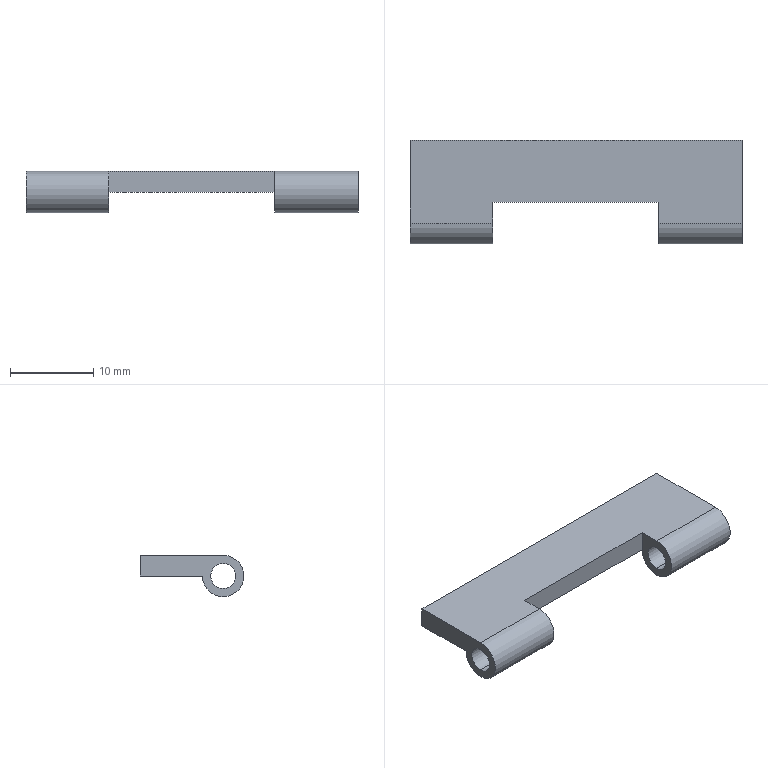Component | SolidWorks | ButtonStation-1_Hinge1-1 | 1 solid | 16 faces | box 40 x 12.5 x 5 mm | volume 1028 mm3 | cylinder 8 | plane 8 | commonest cylinder face diameters 5 x4 3 x4 | material Plain Carbon Steel
STEP:
#1=COLOUR_RGB('',0.7922,0.8196,0.9333);
#2=FILL_AREA_STYLE_COLOUR('',#1);
#3=FILL_AREA_STYLE('',(#2));
#4=SURFACE_STYLE_FILL_AREA(#3);
#5=SURFACE_SIDE_STYLE('',(#4));
#6=SURFACE_STYLE_USAGE(.BOTH.,#5);
#7=PRESENTATION_STYLE_ASSIGNMENT((#6));
#8=CARTESIAN_POINT('',(5.157,24.803,26.811));
#9=VERTEX_POINT('',#8);
#10=CARTESIAN_POINT('',(5.157,24.803,26.614));
#11=VERTEX_POINT('',#10);
#12=CARTESIAN_POINT('',(5.157,24.803,26.713));
#13=DIRECTION('',(1.,-0.,0.));
#14=DIRECTION('',(0.,0.,-1.));
#15=AXIS2_PLACEMENT_3D('',#12,#13,#14);
#16=CIRCLE('',#15,0.09843);
#17=EDGE_CURVE('',#9,#11,#16,.T.);
#18=ORIENTED_EDGE('',*,*,#17,.T.);
#19=CARTESIAN_POINT('',(5.551,24.803,26.614));
#20=VERTEX_POINT('',#19);
#21=CARTESIAN_POINT('',(5.157,24.803,26.614));
#22=DIRECTION('',(1.,-0.,0.));
#23=VECTOR('',#22,39.37);
#24=LINE('',#21,#23);
#25=EDGE_CURVE('',#11,#20,#24,.T.);
#26=ORIENTED_EDGE('',*,*,#25,.T.);
#27=CARTESIAN_POINT('',(5.551,24.803,26.811));
#28=VERTEX_POINT('',#27);
#29=CARTESIAN_POINT('',(5.551,24.803,26.713));
#30=DIRECTION('',(-1.,0.,-0.));
#31=DIRECTION('',(0.,0.,-1.));
#32=AXIS2_PLACEMENT_3D('',#29,#30,#31);
#33=CIRCLE('',#32,0.09843);
#34=EDGE_CURVE('',#20,#28,#33,.T.);
#35=ORIENTED_EDGE('',*,*,#34,.T.);
#36=CARTESIAN_POINT('',(5.157,24.803,26.811));
#37=DIRECTION('',(-1.,0.,-0.));
#38=VECTOR('',#37,39.37);
#39=LINE('',#36,#38);
#40=EDGE_CURVE('',#28,#9,#39,.T.);
#41=ORIENTED_EDGE('',*,*,#40,.T.);
#42=EDGE_LOOP('',(#18,#26,#35,#41));
#43=FACE_OUTER_BOUND('',#42,.T.);
#44=CARTESIAN_POINT('',(5.157,24.803,26.713));
#45=DIRECTION('',(1.,-0.,0.));
#46=DIRECTION('',(0.,0.,-1.));
#47=AXIS2_PLACEMENT_3D('',#44,#45,#46);
#48=CYLINDRICAL_SURFACE('',#47,0.09843);
#49=ADVANCED_FACE('',(#43),#48,.T.);
#50=CARTESIAN_POINT('',(6.339,24.803,26.811));
#51=VERTEX_POINT('',#50);
#52=CARTESIAN_POINT('',(6.339,24.803,26.614));
#53=VERTEX_POINT('',#52);
#54=CARTESIAN_POINT('',(6.339,24.803,26.713));
#55=DIRECTION('',(1.,-0.,0.));
#56=DIRECTION('',(0.,0.,-1.));
#57=AXIS2_PLACEMENT_3D('',#54,#55,#56);
#58=CIRCLE('',#57,0.09843);
#59=EDGE_CURVE('',#51,#53,#58,.T.);
#60=ORIENTED_EDGE('',*,*,#59,.T.);
#61=CARTESIAN_POINT('',(6.732,24.803,26.614));
#62=VERTEX_POINT('',#61);
#63=CARTESIAN_POINT('',(5.157,24.803,26.614));
#64=DIRECTION('',(1.,-0.,0.));
#65=VECTOR('',#64,39.37);
#66=LINE('',#63,#65);
#67=EDGE_CURVE('',#53,#62,#66,.T.);
#68=ORIENTED_EDGE('',*,*,#67,.T.);
#69=CARTESIAN_POINT('',(6.732,24.803,26.811));
#70=VERTEX_POINT('',#69);
#71=CARTESIAN_POINT('',(6.732,24.803,26.713));
#72=DIRECTION('',(-1.,0.,-0.));
#73=DIRECTION('',(0.,0.,-1.));
#74=AXIS2_PLACEMENT_3D('',#71,#72,#73);
#75=CIRCLE('',#74,0.09843);
#76=EDGE_CURVE('',#62,#70,#75,.T.);
#77=ORIENTED_EDGE('',*,*,#76,.T.);
#78=CARTESIAN_POINT('',(5.157,24.803,26.811));
#79=DIRECTION('',(-1.,0.,-0.));
#80=VECTOR('',#79,39.37);
#81=LINE('',#78,#80);
#82=EDGE_CURVE('',#70,#51,#81,.T.);
#83=ORIENTED_EDGE('',*,*,#82,.T.);
#84=EDGE_LOOP('',(#60,#68,#77,#83));
#85=FACE_OUTER_BOUND('',#84,.T.);
#86=CARTESIAN_POINT('',(5.157,24.803,26.713));
#87=DIRECTION('',(1.,-0.,0.));
#88=DIRECTION('',(0.,0.,-1.));
#89=AXIS2_PLACEMENT_3D('',#86,#87,#88);
#90=CYLINDRICAL_SURFACE('',#89,0.09843);
#91=ADVANCED_FACE('',(#85),#90,.T.);
#92=CARTESIAN_POINT('',(5.157,24.803,26.772));
#93=VERTEX_POINT('',#92);
#94=CARTESIAN_POINT('',(5.157,24.803,26.654));
#95=VERTEX_POINT('',#94);
#96=CARTESIAN_POINT('',(5.157,24.803,26.713));
#97=DIRECTION('',(1.,-0.,0.));
#98=DIRECTION('',(0.,0.,-1.));
#99=AXIS2_PLACEMENT_3D('',#96,#97,#98);
#100=CIRCLE('',#99,0.05906);
#101=EDGE_CURVE('',#93,#95,#100,.T.);
#102=ORIENTED_EDGE('',*,*,#101,.F.);
#103=CARTESIAN_POINT('',(5.551,24.803,26.772));
#104=VERTEX_POINT('',#103);
#105=CARTESIAN_POINT('',(5.157,24.803,26.772));
#106=DIRECTION('',(1.,-0.,0.));
#107=VECTOR('',#106,39.37);
#108=LINE('',#105,#107);
#109=EDGE_CURVE('',#93,#104,#108,.T.);
#110=ORIENTED_EDGE('',*,*,#109,.T.);
#111=CARTESIAN_POINT('',(5.551,24.803,26.654));
#112=VERTEX_POINT('',#111);
#113=CARTESIAN_POINT('',(5.551,24.803,26.713));
#114=DIRECTION('',(1.,-0.,0.));
#115=DIRECTION('',(0.,0.,-1.));
#116=AXIS2_PLACEMENT_3D('',#113,#114,#115);
#117=CIRCLE('',#116,0.05906);
#118=EDGE_CURVE('',#104,#112,#117,.T.);
#119=ORIENTED_EDGE('',*,*,#118,.T.);
#120=CARTESIAN_POINT('',(5.157,24.803,26.654));
#121=DIRECTION('',(1.,-0.,0.));
#122=VECTOR('',#121,39.37);
#123=LINE('',#120,#122);
#124=EDGE_CURVE('',#95,#112,#123,.T.);
#125=ORIENTED_EDGE('',*,*,#124,.F.);
#126=EDGE_LOOP('',(#102,#110,#119,#125));
#127=FACE_OUTER_BOUND('',#126,.T.);
#128=CARTESIAN_POINT('',(5.157,24.803,26.713));
#129=DIRECTION('',(1.,-0.,0.));
#130=DIRECTION('',(0.,0.,-1.));
#131=AXIS2_PLACEMENT_3D('',#128,#129,#130);
#132=CYLINDRICAL_SURFACE('',#131,0.05906);
#133=ADVANCED_FACE('',(#127),#132,.F.);
#134=CARTESIAN_POINT('',(6.339,24.803,26.654));
#135=VERTEX_POINT('',#134);
#136=CARTESIAN_POINT('',(6.339,24.803,26.772));
#137=VERTEX_POINT('',#136);
#138=CARTESIAN_POINT('',(6.339,24.803,26.713));
#139=DIRECTION('',(-1.,0.,-0.));
#140=DIRECTION('',(0.,0.,-1.));
#141=AXIS2_PLACEMENT_3D('',#138,#139,#140);
#142=CIRCLE('',#141,0.05906);
#143=EDGE_CURVE('',#135,#137,#142,.T.);
#144=ORIENTED_EDGE('',*,*,#143,.T.);
#145=CARTESIAN_POINT('',(6.732,24.803,26.772));
#146=VERTEX_POINT('',#145);
#147=CARTESIAN_POINT('',(5.157,24.803,26.772));
#148=DIRECTION('',(1.,-0.,0.));
#149=VECTOR('',#148,39.37);
#150=LINE('',#147,#149);
#151=EDGE_CURVE('',#137,#146,#150,.T.);
#152=ORIENTED_EDGE('',*,*,#151,.T.);
#153=CARTESIAN_POINT('',(6.732,24.803,26.654));
#154=VERTEX_POINT('',#153);
#155=CARTESIAN_POINT('',(6.732,24.803,26.713));
#156=DIRECTION('',(1.,-0.,0.));
#157=DIRECTION('',(0.,0.,-1.));
#158=AXIS2_PLACEMENT_3D('',#155,#156,#157);
#159=CIRCLE('',#158,0.05906);
#160=EDGE_CURVE('',#146,#154,#159,.T.);
#161=ORIENTED_EDGE('',*,*,#160,.T.);
#162=CARTESIAN_POINT('',(5.157,24.803,26.654));
#163=DIRECTION('',(1.,-0.,0.));
#164=VECTOR('',#163,39.37);
#165=LINE('',#162,#164);
#166=EDGE_CURVE('',#135,#154,#165,.T.);
#167=ORIENTED_EDGE('',*,*,#166,.F.);
#168=EDGE_LOOP('',(#144,#152,#161,#167));
#169=FACE_OUTER_BOUND('',#168,.T.);
#170=CARTESIAN_POINT('',(5.157,24.803,26.713));
#171=DIRECTION('',(1.,-0.,0.));
#172=DIRECTION('',(0.,0.,-1.));
#173=AXIS2_PLACEMENT_3D('',#170,#171,#172);
#174=CYLINDRICAL_SURFACE('',#173,0.05906);
#175=ADVANCED_FACE('',(#169),#174,.F.);
#176=CARTESIAN_POINT('',(5.551,24.902,26.811));
#177=VERTEX_POINT('',#176);
#178=CARTESIAN_POINT('',(5.551,24.932,26.811));
#179=DIRECTION('',(-0.,-1.,0.));
#180=VECTOR('',#179,39.37);
#181=LINE('',#178,#180);
#182=EDGE_CURVE('',#177,#28,#181,.T.);
#183=ORIENTED_EDGE('',*,*,#182,.F.);
#184=CARTESIAN_POINT('',(6.339,24.902,26.811));
#185=VERTEX_POINT('',#184);
#186=CARTESIAN_POINT('',(5.157,24.902,26.811));
#187=DIRECTION('',(-1.,0.,-0.));
#188=VECTOR('',#187,39.37);
#189=LINE('',#186,#188);
#190=EDGE_CURVE('',#185,#177,#189,.T.);
#191=ORIENTED_EDGE('',*,*,#190,.F.);
#192=CARTESIAN_POINT('',(6.339,24.932,26.811));
#193=DIRECTION('',(0.,1.,-0.));
#194=VECTOR('',#193,39.37);
#195=LINE('',#192,#194);
#196=EDGE_CURVE('',#51,#185,#195,.T.);
#197=ORIENTED_EDGE('',*,*,#196,.F.);
#198=ORIENTED_EDGE('',*,*,#82,.F.);
#199=CARTESIAN_POINT('',(6.732,25.197,26.811));
#200=VERTEX_POINT('',#199);
#201=CARTESIAN_POINT('',(6.732,24.932,26.811));
#202=DIRECTION('',(-0.,-1.,0.));
#203=VECTOR('',#202,39.37);
#204=LINE('',#201,#203);
#205=EDGE_CURVE('',#200,#70,#204,.T.);
#206=ORIENTED_EDGE('',*,*,#205,.F.);
#207=CARTESIAN_POINT('',(5.157,25.197,26.811));
#208=VERTEX_POINT('',#207);
#209=CARTESIAN_POINT('',(5.157,25.197,26.811));
#210=DIRECTION('',(1.,-0.,0.));
#211=VECTOR('',#210,39.37);
#212=LINE('',#209,#211);
#213=EDGE_CURVE('',#208,#200,#212,.T.);
#214=ORIENTED_EDGE('',*,*,#213,.F.);
#215=CARTESIAN_POINT('',(5.157,24.932,26.811));
#216=DIRECTION('',(0.,1.,-0.));
#217=VECTOR('',#216,39.37);
#218=LINE('',#215,#217);
#219=EDGE_CURVE('',#9,#208,#218,.T.);
#220=ORIENTED_EDGE('',*,*,#219,.F.);
#221=ORIENTED_EDGE('',*,*,#40,.F.);
#222=EDGE_LOOP('',(#183,#191,#197,#198,#206,#214,#220,#221));
#223=FACE_OUTER_BOUND('',#222,.T.);
#224=CARTESIAN_POINT('',(5.157,24.932,26.811));
#225=DIRECTION('',(0.,-0.,-1.));
#226=DIRECTION('',(-1.,0.,-0.));
#227=AXIS2_PLACEMENT_3D('',#224,#225,#226);
#228=PLANE('',#227);
#229=ADVANCED_FACE('',(#223),#228,.F.);
#230=ORIENTED_EDGE('',*,*,#25,.F.);
#231=CARTESIAN_POINT('',(5.157,24.902,26.713));
#232=VERTEX_POINT('',#231);
#233=CARTESIAN_POINT('',(5.157,24.803,26.713));
#234=DIRECTION('',(1.,-0.,0.));
#235=DIRECTION('',(0.,0.,-1.));
#236=AXIS2_PLACEMENT_3D('',#233,#234,#235);
#237=CIRCLE('',#236,0.09843);
#238=EDGE_CURVE('',#11,#232,#237,.T.);
#239=ORIENTED_EDGE('',*,*,#238,.T.);
#240=CARTESIAN_POINT('',(5.551,24.902,26.713));
#241=VERTEX_POINT('',#240);
#242=CARTESIAN_POINT('',(5.157,24.902,26.713));
#243=DIRECTION('',(1.,-0.,0.));
#244=VECTOR('',#243,39.37);
#245=LINE('',#242,#244);
#246=EDGE_CURVE('',#232,#241,#245,.T.);
#247=ORIENTED_EDGE('',*,*,#246,.T.);
#248=CARTESIAN_POINT('',(5.551,24.803,26.713));
#249=DIRECTION('',(-1.,0.,-0.));
#250=DIRECTION('',(0.,0.,-1.));
#251=AXIS2_PLACEMENT_3D('',#248,#249,#250);
#252=CIRCLE('',#251,0.09843);
#253=EDGE_CURVE('',#241,#20,#252,.T.);
#254=ORIENTED_EDGE('',*,*,#253,.T.);
#255=EDGE_LOOP('',(#230,#239,#247,#254));
#256=FACE_OUTER_BOUND('',#255,.T.);
#257=CARTESIAN_POINT('',(5.157,24.803,26.713));
#258=DIRECTION('',(1.,-0.,0.));
#259=DIRECTION('',(0.,0.,-1.));
#260=AXIS2_PLACEMENT_3D('',#257,#258,#259);
#261=CYLINDRICAL_SURFACE('',#260,0.09843);
#262=ADVANCED_FACE('',(#256),#261,.T.);
#263=CARTESIAN_POINT('',(5.551,24.803,26.713));
#264=DIRECTION('',(1.,-0.,0.));
#265=DIRECTION('',(0.,0.,-1.));
#266=AXIS2_PLACEMENT_3D('',#263,#264,#265);
#267=CIRCLE('',#266,0.05906);
#268=EDGE_CURVE('',#112,#104,#267,.T.);
#269=ORIENTED_EDGE('',*,*,#268,.F.);
#270=ORIENTED_EDGE('',*,*,#118,.F.);
#271=EDGE_LOOP('',(#269,#270));
#272=FACE_BOUND('',#271,.T.);
#273=ORIENTED_EDGE('',*,*,#253,.F.);
#274=CARTESIAN_POINT('',(5.551,24.902,26.614));
#275=DIRECTION('',(0.,-0.,-1.));
#276=VECTOR('',#275,39.37);
#277=LINE('',#274,#276);
#278=EDGE_CURVE('',#177,#241,#277,.T.);
#279=ORIENTED_EDGE('',*,*,#278,.F.);
#280=ORIENTED_EDGE('',*,*,#182,.T.);
#281=ORIENTED_EDGE('',*,*,#34,.F.);
#282=EDGE_LOOP('',(#273,#279,#280,#281));
#283=FACE_OUTER_BOUND('',#282,.T.);
#284=CARTESIAN_POINT('',(5.551,24.705,26.614));
#285=DIRECTION('',(-1.,0.,-0.));
#286=DIRECTION('',(-0.,0.,1.));
#287=AXIS2_PLACEMENT_3D('',#284,#285,#286);
#288=PLANE('',#287);
#289=ADVANCED_FACE('',(#272,#283),#288,.F.);
#290=CARTESIAN_POINT('',(6.339,24.902,26.713));
#291=VERTEX_POINT('',#290);
#292=CARTESIAN_POINT('',(6.339,24.902,26.614));
#293=DIRECTION('',(0.,-0.,-1.));
#294=VECTOR('',#293,39.37);
#295=LINE('',#292,#294);
#296=EDGE_CURVE('',#185,#291,#295,.T.);
#297=ORIENTED_EDGE('',*,*,#296,.F.);
#298=ORIENTED_EDGE('',*,*,#190,.T.);
#299=ORIENTED_EDGE('',*,*,#278,.T.);
#300=CARTESIAN_POINT('',(5.551,24.902,26.713));
#301=DIRECTION('',(-1.,0.,-0.));
#302=VECTOR('',#301,39.37);
#303=LINE('',#300,#302);
#304=EDGE_CURVE('',#291,#241,#303,.T.);
#305=ORIENTED_EDGE('',*,*,#304,.F.);
#306=EDGE_LOOP('',(#297,#298,#299,#305));
#307=FACE_OUTER_BOUND('',#306,.T.);
#308=CARTESIAN_POINT('',(5.551,24.902,26.614));
#309=DIRECTION('',(0.,1.,-0.));
#310=DIRECTION('',(0.,-0.,-1.));
#311=AXIS2_PLACEMENT_3D('',#308,#309,#310);
#312=PLANE('',#311);
#313=ADVANCED_FACE('',(#307),#312,.F.);
#314=ORIENTED_EDGE('',*,*,#143,.F.);
#315=CARTESIAN_POINT('',(6.339,24.803,26.713));
#316=DIRECTION('',(-1.,0.,-0.));
#317=DIRECTION('',(0.,0.,-1.));
#318=AXIS2_PLACEMENT_3D('',#315,#316,#317);
#319=CIRCLE('',#318,0.05906);
#320=EDGE_CURVE('',#137,#135,#319,.T.);
#321=ORIENTED_EDGE('',*,*,#320,.F.);
#322=EDGE_LOOP('',(#314,#321));
#323=FACE_BOUND('',#322,.T.);
#324=ORIENTED_EDGE('',*,*,#59,.F.);
#325=ORIENTED_EDGE('',*,*,#196,.T.);
#326=ORIENTED_EDGE('',*,*,#296,.T.);
#327=CARTESIAN_POINT('',(6.339,24.803,26.713));
#328=DIRECTION('',(1.,-0.,0.));
#329=DIRECTION('',(0.,0.,-1.));
#330=AXIS2_PLACEMENT_3D('',#327,#328,#329);
#331=CIRCLE('',#330,0.09843);
#332=EDGE_CURVE('',#53,#291,#331,.T.);
#333=ORIENTED_EDGE('',*,*,#332,.F.);
#334=EDGE_LOOP('',(#324,#325,#326,#333));
#335=FACE_OUTER_BOUND('',#334,.T.);
#336=CARTESIAN_POINT('',(6.339,24.705,26.614));
#337=DIRECTION('',(1.,-0.,0.));
#338=DIRECTION('',(0.,-0.,-1.));
#339=AXIS2_PLACEMENT_3D('',#336,#337,#338);
#340=PLANE('',#339);
#341=ADVANCED_FACE('',(#323,#335),#340,.F.);
#342=ORIENTED_EDGE('',*,*,#67,.F.);
#343=ORIENTED_EDGE('',*,*,#332,.T.);
#344=CARTESIAN_POINT('',(6.732,24.902,26.713));
#345=VERTEX_POINT('',#344);
#346=CARTESIAN_POINT('',(5.157,24.902,26.713));
#347=DIRECTION('',(-1.,0.,-0.));
#348=VECTOR('',#347,39.37);
#349=LINE('',#346,#348);
#350=EDGE_CURVE('',#345,#291,#349,.T.);
#351=ORIENTED_EDGE('',*,*,#350,.F.);
#352=CARTESIAN_POINT('',(6.732,24.803,26.713));
#353=DIRECTION('',(-1.,0.,-0.));
#354=DIRECTION('',(0.,0.,-1.));
#355=AXIS2_PLACEMENT_3D('',#352,#353,#354);
#356=CIRCLE('',#355,0.09843);
#357=EDGE_CURVE('',#345,#62,#356,.T.);
#358=ORIENTED_EDGE('',*,*,#357,.T.);
#359=EDGE_LOOP('',(#342,#343,#351,#358));
#360=FACE_OUTER_BOUND('',#359,.T.);
#361=CARTESIAN_POINT('',(5.157,24.803,26.713));
#362=DIRECTION('',(1.,-0.,0.));
#363=DIRECTION('',(0.,0.,-1.));
#364=AXIS2_PLACEMENT_3D('',#361,#362,#363);
#365=CYLINDRICAL_SURFACE('',#364,0.09843);
#366=ADVANCED_FACE('',(#360),#365,.T.);
#367=CARTESIAN_POINT('',(6.732,24.803,26.713));
#368=DIRECTION('',(1.,-0.,0.));
#369=DIRECTION('',(0.,0.,-1.));
#370=AXIS2_PLACEMENT_3D('',#367,#368,#369);
#371=CIRCLE('',#370,0.05906);
#372=EDGE_CURVE('',#154,#146,#371,.T.);
#373=ORIENTED_EDGE('',*,*,#372,.F.);
#374=ORIENTED_EDGE('',*,*,#160,.F.);
#375=EDGE_LOOP('',(#373,#374));
#376=FACE_BOUND('',#375,.T.);
#377=ORIENTED_EDGE('',*,*,#357,.F.);
#378=CARTESIAN_POINT('',(6.732,25.197,26.713));
#379=VERTEX_POINT('',#378);
#380=CARTESIAN_POINT('',(6.732,24.932,26.713));
#381=DIRECTION('',(-0.,-1.,0.));
#382=VECTOR('',#381,39.37);
#383=LINE('',#380,#382);
#384=EDGE_CURVE('',#379,#345,#383,.T.);
#385=ORIENTED_EDGE('',*,*,#384,.F.);
#386=CARTESIAN_POINT('',(6.732,25.197,27.174));
#387=DIRECTION('',(0.,-0.,-1.));
#388=VECTOR('',#387,39.37);
#389=LINE('',#386,#388);
#390=EDGE_CURVE('',#200,#379,#389,.T.);
#391=ORIENTED_EDGE('',*,*,#390,.F.);
#392=ORIENTED_EDGE('',*,*,#205,.T.);
#393=ORIENTED_EDGE('',*,*,#76,.F.);
#394=EDGE_LOOP('',(#377,#385,#391,#392,#393));
#395=FACE_OUTER_BOUND('',#394,.T.);
#396=CARTESIAN_POINT('',(6.732,24.932,27.174));
#397=DIRECTION('',(-1.,0.,-0.));
#398=DIRECTION('',(-0.,0.,1.));
#399=AXIS2_PLACEMENT_3D('',#396,#397,#398);
#400=PLANE('',#399);
#401=ADVANCED_FACE('',(#376,#395),#400,.F.);
#402=CARTESIAN_POINT('',(5.157,25.197,26.713));
#403=VERTEX_POINT('',#402);
#404=CARTESIAN_POINT('',(5.157,25.197,27.174));
#405=DIRECTION('',(-0.,0.,1.));
#406=VECTOR('',#405,39.37);
#407=LINE('',#404,#406);
#408=EDGE_CURVE('',#403,#208,#407,.T.);
#409=ORIENTED_EDGE('',*,*,#408,.T.);
#410=ORIENTED_EDGE('',*,*,#213,.T.);
#411=ORIENTED_EDGE('',*,*,#390,.T.);
#412=CARTESIAN_POINT('',(5.157,25.197,26.713));
#413=DIRECTION('',(-1.,0.,-0.));
#414=VECTOR('',#413,39.37);
#415=LINE('',#412,#414);
#416=EDGE_CURVE('',#379,#403,#415,.T.);
#417=ORIENTED_EDGE('',*,*,#416,.T.);
#418=EDGE_LOOP('',(#409,#410,#411,#417));
#419=FACE_OUTER_BOUND('',#418,.T.);
#420=CARTESIAN_POINT('',(5.157,25.197,27.174));
#421=DIRECTION('',(0.,1.,-0.));
#422=DIRECTION('',(0.,-0.,-1.));
#423=AXIS2_PLACEMENT_3D('',#420,#421,#422);
#424=PLANE('',#423);
#425=ADVANCED_FACE('',(#419),#424,.T.);
#426=CARTESIAN_POINT('',(5.157,24.803,26.713));
#427=DIRECTION('',(1.,-0.,0.));
#428=DIRECTION('',(0.,0.,-1.));
#429=AXIS2_PLACEMENT_3D('',#426,#427,#428);
#430=CIRCLE('',#429,0.05906);
#431=EDGE_CURVE('',#95,#93,#430,.T.);
#432=ORIENTED_EDGE('',*,*,#431,.T.);
#433=ORIENTED_EDGE('',*,*,#101,.T.);
#434=EDGE_LOOP('',(#432,#433));
#435=FACE_BOUND('',#434,.T.);
#436=CARTESIAN_POINT('',(5.157,24.932,26.713));
#437=DIRECTION('',(-0.,-1.,0.));
#438=VECTOR('',#437,39.37);
#439=LINE('',#436,#438);
#440=EDGE_CURVE('',#403,#232,#439,.T.);
#441=ORIENTED_EDGE('',*,*,#440,.T.);
#442=ORIENTED_EDGE('',*,*,#238,.F.);
#443=ORIENTED_EDGE('',*,*,#17,.F.);
#444=ORIENTED_EDGE('',*,*,#219,.T.);
#445=ORIENTED_EDGE('',*,*,#408,.F.);
#446=EDGE_LOOP('',(#441,#442,#443,#444,#445));
#447=FACE_OUTER_BOUND('',#446,.T.);
#448=CARTESIAN_POINT('',(5.157,24.932,27.174));
#449=DIRECTION('',(-1.,0.,-0.));
#450=DIRECTION('',(-0.,0.,1.));
#451=AXIS2_PLACEMENT_3D('',#448,#449,#450);
#452=PLANE('',#451);
#453=ADVANCED_FACE('',(#435,#447),#452,.T.);
#454=ORIENTED_EDGE('',*,*,#109,.F.);
#455=ORIENTED_EDGE('',*,*,#431,.F.);
#456=ORIENTED_EDGE('',*,*,#124,.T.);
#457=ORIENTED_EDGE('',*,*,#268,.T.);
#458=EDGE_LOOP('',(#454,#455,#456,#457));
#459=FACE_OUTER_BOUND('',#458,.T.);
#460=CARTESIAN_POINT('',(5.157,24.803,26.713));
#461=DIRECTION('',(1.,-0.,0.));
#462=DIRECTION('',(0.,0.,-1.));
#463=AXIS2_PLACEMENT_3D('',#460,#461,#462);
#464=CYLINDRICAL_SURFACE('',#463,0.05906);
#465=ADVANCED_FACE('',(#459),#464,.F.);
#466=ORIENTED_EDGE('',*,*,#440,.F.);
#467=ORIENTED_EDGE('',*,*,#416,.F.);
#468=ORIENTED_EDGE('',*,*,#384,.T.);
#469=ORIENTED_EDGE('',*,*,#350,.T.);
#470=ORIENTED_EDGE('',*,*,#304,.T.);
#471=ORIENTED_EDGE('',*,*,#246,.F.);
#472=EDGE_LOOP('',(#466,#467,#468,#469,#470,#471));
#473=FACE_OUTER_BOUND('',#472,.T.);
#474=CARTESIAN_POINT('',(5.157,24.932,26.713));
#475=DIRECTION('',(0.,-0.,-1.));
#476=DIRECTION('',(-1.,0.,-0.));
#477=AXIS2_PLACEMENT_3D('',#474,#475,#476);
#478=PLANE('',#477);
#479=ADVANCED_FACE('',(#473),#478,.T.);
#480=ORIENTED_EDGE('',*,*,#151,.F.);
#481=ORIENTED_EDGE('',*,*,#320,.T.);
#482=ORIENTED_EDGE('',*,*,#166,.T.);
#483=ORIENTED_EDGE('',*,*,#372,.T.);
#484=EDGE_LOOP('',(#480,#481,#482,#483));
#485=FACE_OUTER_BOUND('',#484,.T.);
#486=CARTESIAN_POINT('',(5.157,24.803,26.713));
#487=DIRECTION('',(1.,-0.,0.));
#488=DIRECTION('',(0.,0.,-1.));
#489=AXIS2_PLACEMENT_3D('',#486,#487,#488);
#490=CYLINDRICAL_SURFACE('',#489,0.05906);
#491=ADVANCED_FACE('',(#485),#490,.F.);
#492=CLOSED_SHELL('',(#49,#91,#133,#175,#229,#262,#289,#313,#341,#366,#401,#425,#453,#465,#479,#491));
#493=MANIFOLD_SOLID_BREP('',#492);
#494=STYLED_ITEM('',(#7),#493);
#495=(LENGTH_UNIT()NAMED_UNIT(*)SI_UNIT($,.METRE.));
#496=LENGTH_MEASURE_WITH_UNIT(LENGTH_MEASURE(0.0254),#495);
#497=DIMENSIONAL_EXPONENTS(1.,0.,0.,0.,0.,0.,0.);
#498=(CONVERSION_BASED_UNIT('',#496)LENGTH_UNIT()NAMED_UNIT(#497));
#499=UNCERTAINTY_MEASURE_WITH_UNIT(LENGTH_MEASURE(0.00001),#498,'','');
#500=(NAMED_UNIT(*)PLANE_ANGLE_UNIT()SI_UNIT($,.RADIAN.));
#501=(NAMED_UNIT(*)SI_UNIT($,.STERADIAN.)SOLID_ANGLE_UNIT());
#502=(GEOMETRIC_REPRESENTATION_CONTEXT(3)GLOBAL_UNCERTAINTY_ASSIGNED_CONTEXT((#499))GLOBAL_UNIT_ASSIGNED_CONTEXT((#498,#500,#501))REPRESENTATION_CONTEXT('',''));
#503=MECHANICAL_DESIGN_GEOMETRIC_PRESENTATION_REPRESENTATION('',(#494),#502);
#504=PRESENTATION_LAYER_ASSIGNMENT('','',(#494));
#505=CARTESIAN_POINT('',(0.,0.,0.));
#506=DIRECTION('',(0.,0.,1.));
#507=DIRECTION('',(1.,0.,0.));
#508=AXIS2_PLACEMENT_3D('',#505,#506,#507);
#509=(LENGTH_UNIT()NAMED_UNIT(*)SI_UNIT($,.METRE.));
#510=LENGTH_MEASURE_WITH_UNIT(LENGTH_MEASURE(0.0254),#509);
#511=DIMENSIONAL_EXPONENTS(1.,0.,0.,0.,0.,0.,0.);
#512=(CONVERSION_BASED_UNIT('',#510)LENGTH_UNIT()NAMED_UNIT(#511));
#513=UNCERTAINTY_MEASURE_WITH_UNIT(LENGTH_MEASURE(0.00001),#512,'','');
#514=(NAMED_UNIT(*)PLANE_ANGLE_UNIT()SI_UNIT($,.RADIAN.));
#515=(NAMED_UNIT(*)SI_UNIT($,.STERADIAN.)SOLID_ANGLE_UNIT());
#516=(GEOMETRIC_REPRESENTATION_CONTEXT(3)GLOBAL_UNCERTAINTY_ASSIGNED_CONTEXT((#513))GLOBAL_UNIT_ASSIGNED_CONTEXT((#512,#514,#515))REPRESENTATION_CONTEXT('',''));
#517=ADVANCED_BREP_SHAPE_REPRESENTATION('',(#493,#508),#516);